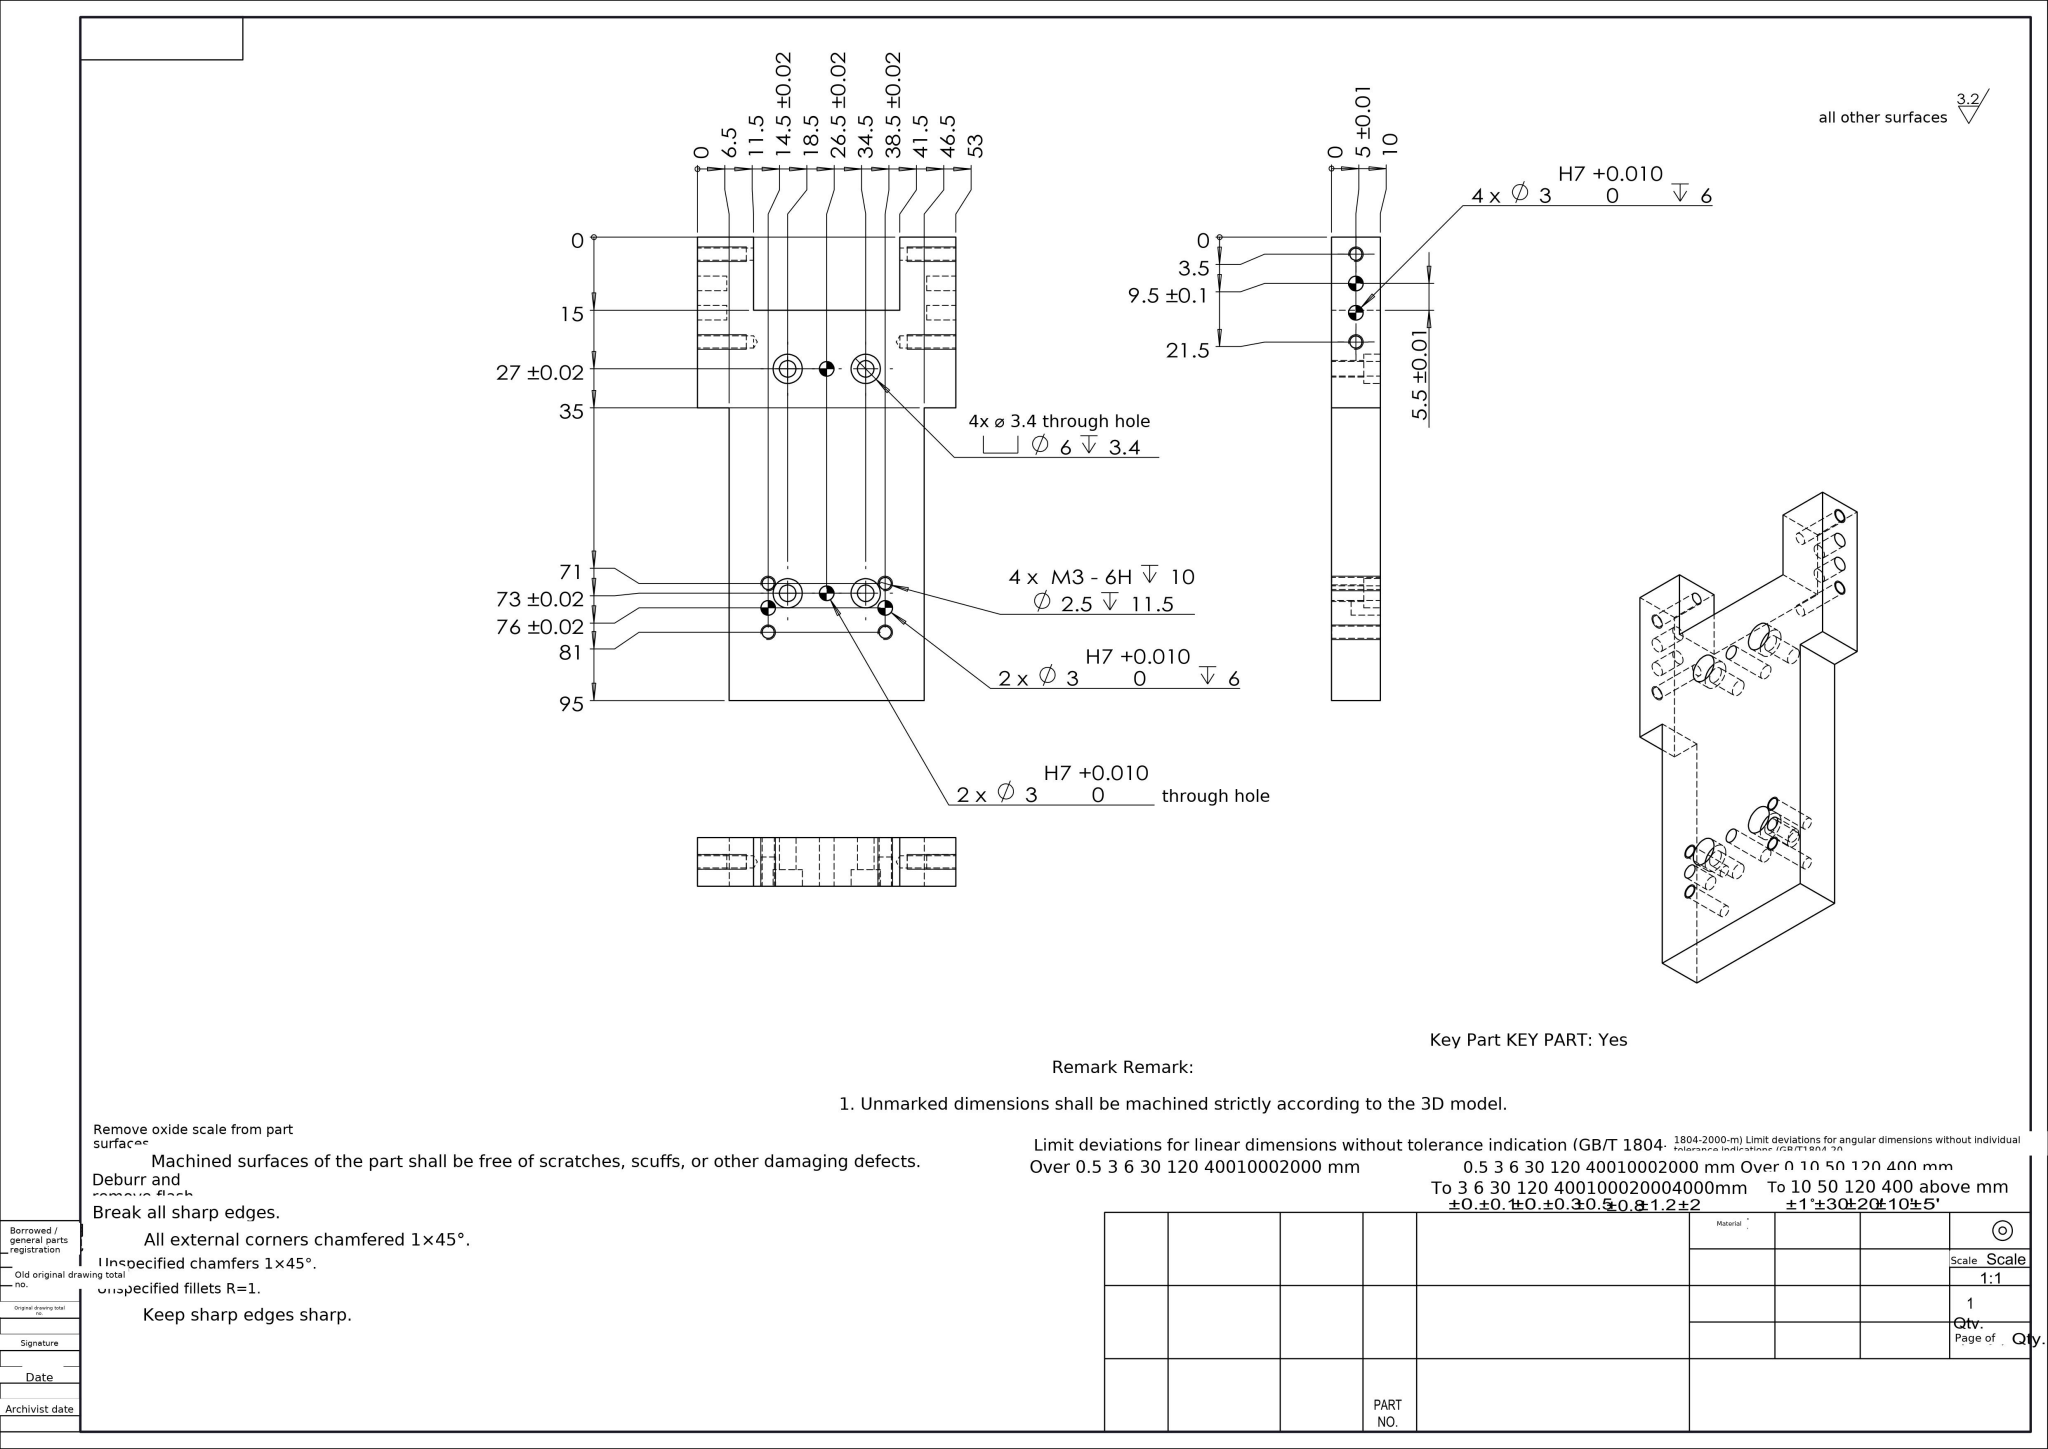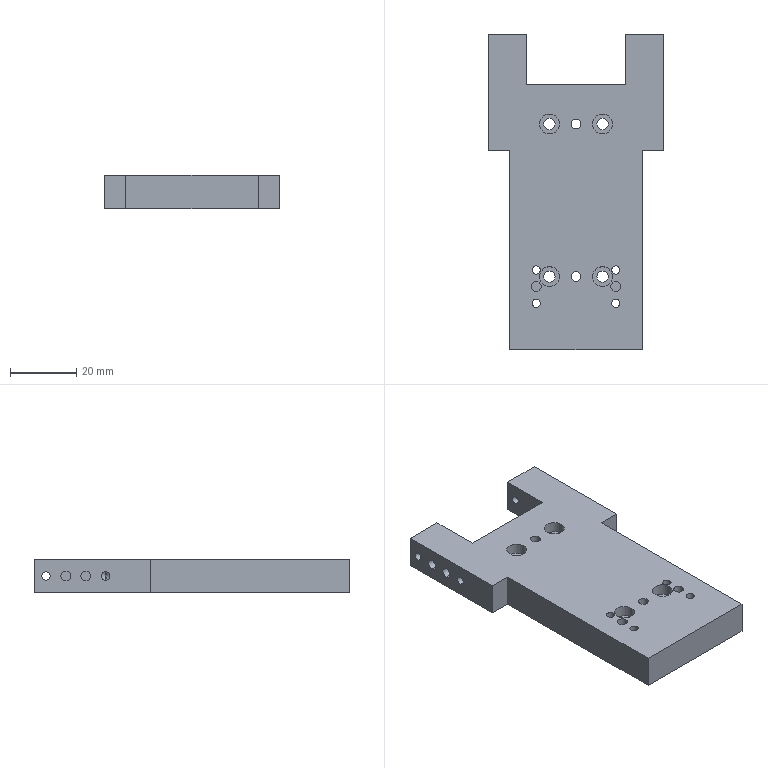Part | SolidWorks | mm | 1 solid | 76 faces | box 53 x 95 x 10 mm | volume 36605 mm3 | cylinder 48 | plane 24 | cone 4 | commonest cylinder face diameters 3 x16 2.5 x16 6 x8 3.4 x8
build123d program:
from build123d import *

# Parameters (mm, degrees)
SKETCH1_W                                         = 40
SKETCH1_H                                         = 95
BOSS_EXTRUDE1_DEPTH                               = 10
SKETCH2_W                                         = 53
SKETCH2_H                                         = 10
BOSS_EXTRUDE2_DEPTH                               = 35
M3_TAPPED_HOLE1_AT_2_COUNT                        = 2
M3_TAPPED_HOLE1_AT_2_PITCH                        = 18
SIZE_MM_DOWEL_PIN_HOLE1_D                         = 3
SIZE_MM_DOWEL_PIN_HOLE1_DEPTH                     = 6
HOLE_SIZE_ACCORDING_TO_HEXAGON_SOCKET_D           = 3.4
HOLE_SIZE_ACCORDING_TO_HEXAGON_SOCKET_CBORE_D     = 6
HOLE_SIZE_ACCORDING_TO_HEXAGON_SOCKET_CBORE_DEPTH = 3.4
SIZE_MM_DOWEL_PIN_HOLE2_D                         = 3
M3_TAPPED_HOLE2_D                                 = 2.5
M3_TAPPED_HOLE2_DEPTH                             = 11.5
M3_TAPPED_HOLE2_TIP                               = 0.7511
SIZE_MM_DOWEL_PIN_HOLE3_D                         = 3
SIZE_MM_DOWEL_PIN_HOLE3_DEPTH                     = 6
CUT_EXTRUDE1_REACH                                = 57.304
SKETCH15_W                                        = 30
SKETCH15_H                                        = 30


with BuildPart() as part:
    # Sketch1 → Boss-Extrude1 (new body)
    with BuildSketch(Plane.XY):
        Rectangle(SKETCH1_W, SKETCH1_H)
    extrude(amount=BOSS_EXTRUDE1_DEPTH)

    # Sketch2 → Boss-Extrude2 (add)
    with BuildSketch(Plane(origin=(0, 47.5, 0), x_dir=(1, 0, 0), z_dir=(0, 1, 0))):
        with Locations((0, -5)):
            Rectangle(SKETCH2_W, SKETCH2_H)
    extrude(amount=-BOSS_EXTRUDE2_DEPTH)

    # Sketch4 → M3 Tapped Hole1 (revolve, cut)
    with BuildSketch(Plane(origin=(-26.5, 26, 5), x_dir=(0, 0, 1), z_dir=(0, 1, 0))):
        Polygon((0, 0), (0, 12.251), (1.25, 11.5), (1.25, 0), align=None)
    m3_tapped_hole1 = revolve(axis=Axis((-32.85, 26, 5), (1, 0, 0)), mode=Mode.SUBTRACT)

    # M3 Tapped Hole1 at 2: M3 Tapped Hole1 ×2
    with Locations(*[(0, i * M3_TAPPED_HOLE1_AT_2_PITCH, 0) for i in range(1, M3_TAPPED_HOLE1_AT_2_COUNT)]):
        add(m3_tapped_hole1, mode=Mode.SUBTRACT)

    # Size mm Dowel Pin Hole1
    with Locations(Plane.ZY.offset(26.5)):
        with Locations((5, 38), (5, 32)):
            size_mm_dowel_pin_hole1 = Hole(SIZE_MM_DOWEL_PIN_HOLE1_D / 2, depth=SIZE_MM_DOWEL_PIN_HOLE1_DEPTH)

    # Mirror1: M3 Tapped Hole1, Size mm Dowel Pin Hole1 across plane
    add(m3_tapped_hole1.mirror(Plane(origin=(0, 0, 0), x_dir=(0, 0, 1), z_dir=(1, 0, 0))), mode=Mode.SUBTRACT)
    add(size_mm_dowel_pin_hole1.mirror(Plane(origin=(0, 0, 0), x_dir=(0, 0, 1), z_dir=(1, 0, 0))), mode=Mode.SUBTRACT)

    # Mirror1 copy 1 sketch → Mirror1 copy 1 (revolve, cut)
    with BuildSketch(Plane(origin=(26.5, 44, 5), x_dir=(0, 0, 1), z_dir=(0, 1, 0))):
        Polygon((0, 0), (0, -12.251), (1.25, -11.5), (1.25, 0), align=None)
    revolve(axis=Axis((32.85, 44, 5), (1, 0, 0)), mode=Mode.SUBTRACT)

    # Hole Size _ according to_ Hexagon Socket (through all)
    with Locations(Plane.XY.offset(10)):
        with Locations((8, 20.5), (-8, 20.5), (8, -25.5), (-8, -25.5)):
            CounterBoreHole(HOLE_SIZE_ACCORDING_TO_HEXAGON_SOCKET_D / 2, HOLE_SIZE_ACCORDING_TO_HEXAGON_SOCKET_CBORE_D / 2, HOLE_SIZE_ACCORDING_TO_HEXAGON_SOCKET_CBORE_DEPTH)

    # Size mm Dowel Pin Hole2 (through all)
    with Locations(Plane.XY.offset(10)):
        with Locations((0, 20.5), (0, -25.5)):
            Hole(SIZE_MM_DOWEL_PIN_HOLE2_D / 2)

    # M3 Tapped Hole2
    with Locations(Plane.XY.offset(10)):
        with Locations((12, -33.5), (-12, -33.5), (12, -23.5), (-12, -23.5)):
            Hole(M3_TAPPED_HOLE2_D / 2, depth=M3_TAPPED_HOLE2_DEPTH)
            with Locations((0, 0, -(M3_TAPPED_HOLE2_DEPTH + M3_TAPPED_HOLE2_TIP / 2))):  # 118° drill point
                Cone(0, M3_TAPPED_HOLE2_D / 2, M3_TAPPED_HOLE2_TIP, mode=Mode.SUBTRACT)

    # Size mm Dowel Pin Hole3
    with Locations(Plane.XY.offset(10)):
        with Locations((12, -28.5), (-12, -28.5)):
            Hole(SIZE_MM_DOWEL_PIN_HOLE3_D / 2, depth=SIZE_MM_DOWEL_PIN_HOLE3_DEPTH)

    # Cut-Extrude1: up to this face of the body (flat: up to its plane)
    cut_extrude1_end = Plane(part.part.faces().sort_by_distance((0, 3.426, 0))[0])
    # Sketch15 → Cut-Extrude1 (cut, up to the picked face)
    with BuildSketch(Plane.XY.offset(10), mode=Mode.PRIVATE) as cut_extrude1_sk1:
        with Locations((0, 47.5)):
            Rectangle(SKETCH15_W, SKETCH15_H)
    cut_extrude1_tool1 = split(extrude(cut_extrude1_sk1.sketch, amount=-CUT_EXTRUDE1_REACH, mode=Mode.PRIVATE), bisect_by=cut_extrude1_end, keep=Keep.BOTH, mode=Mode.PRIVATE)
    add(cut_extrude1_tool1.solids().sort_by(Axis((0, 47.5, 10), (0, 0, -1)))[0], mode=Mode.SUBTRACT)


solid = part.part